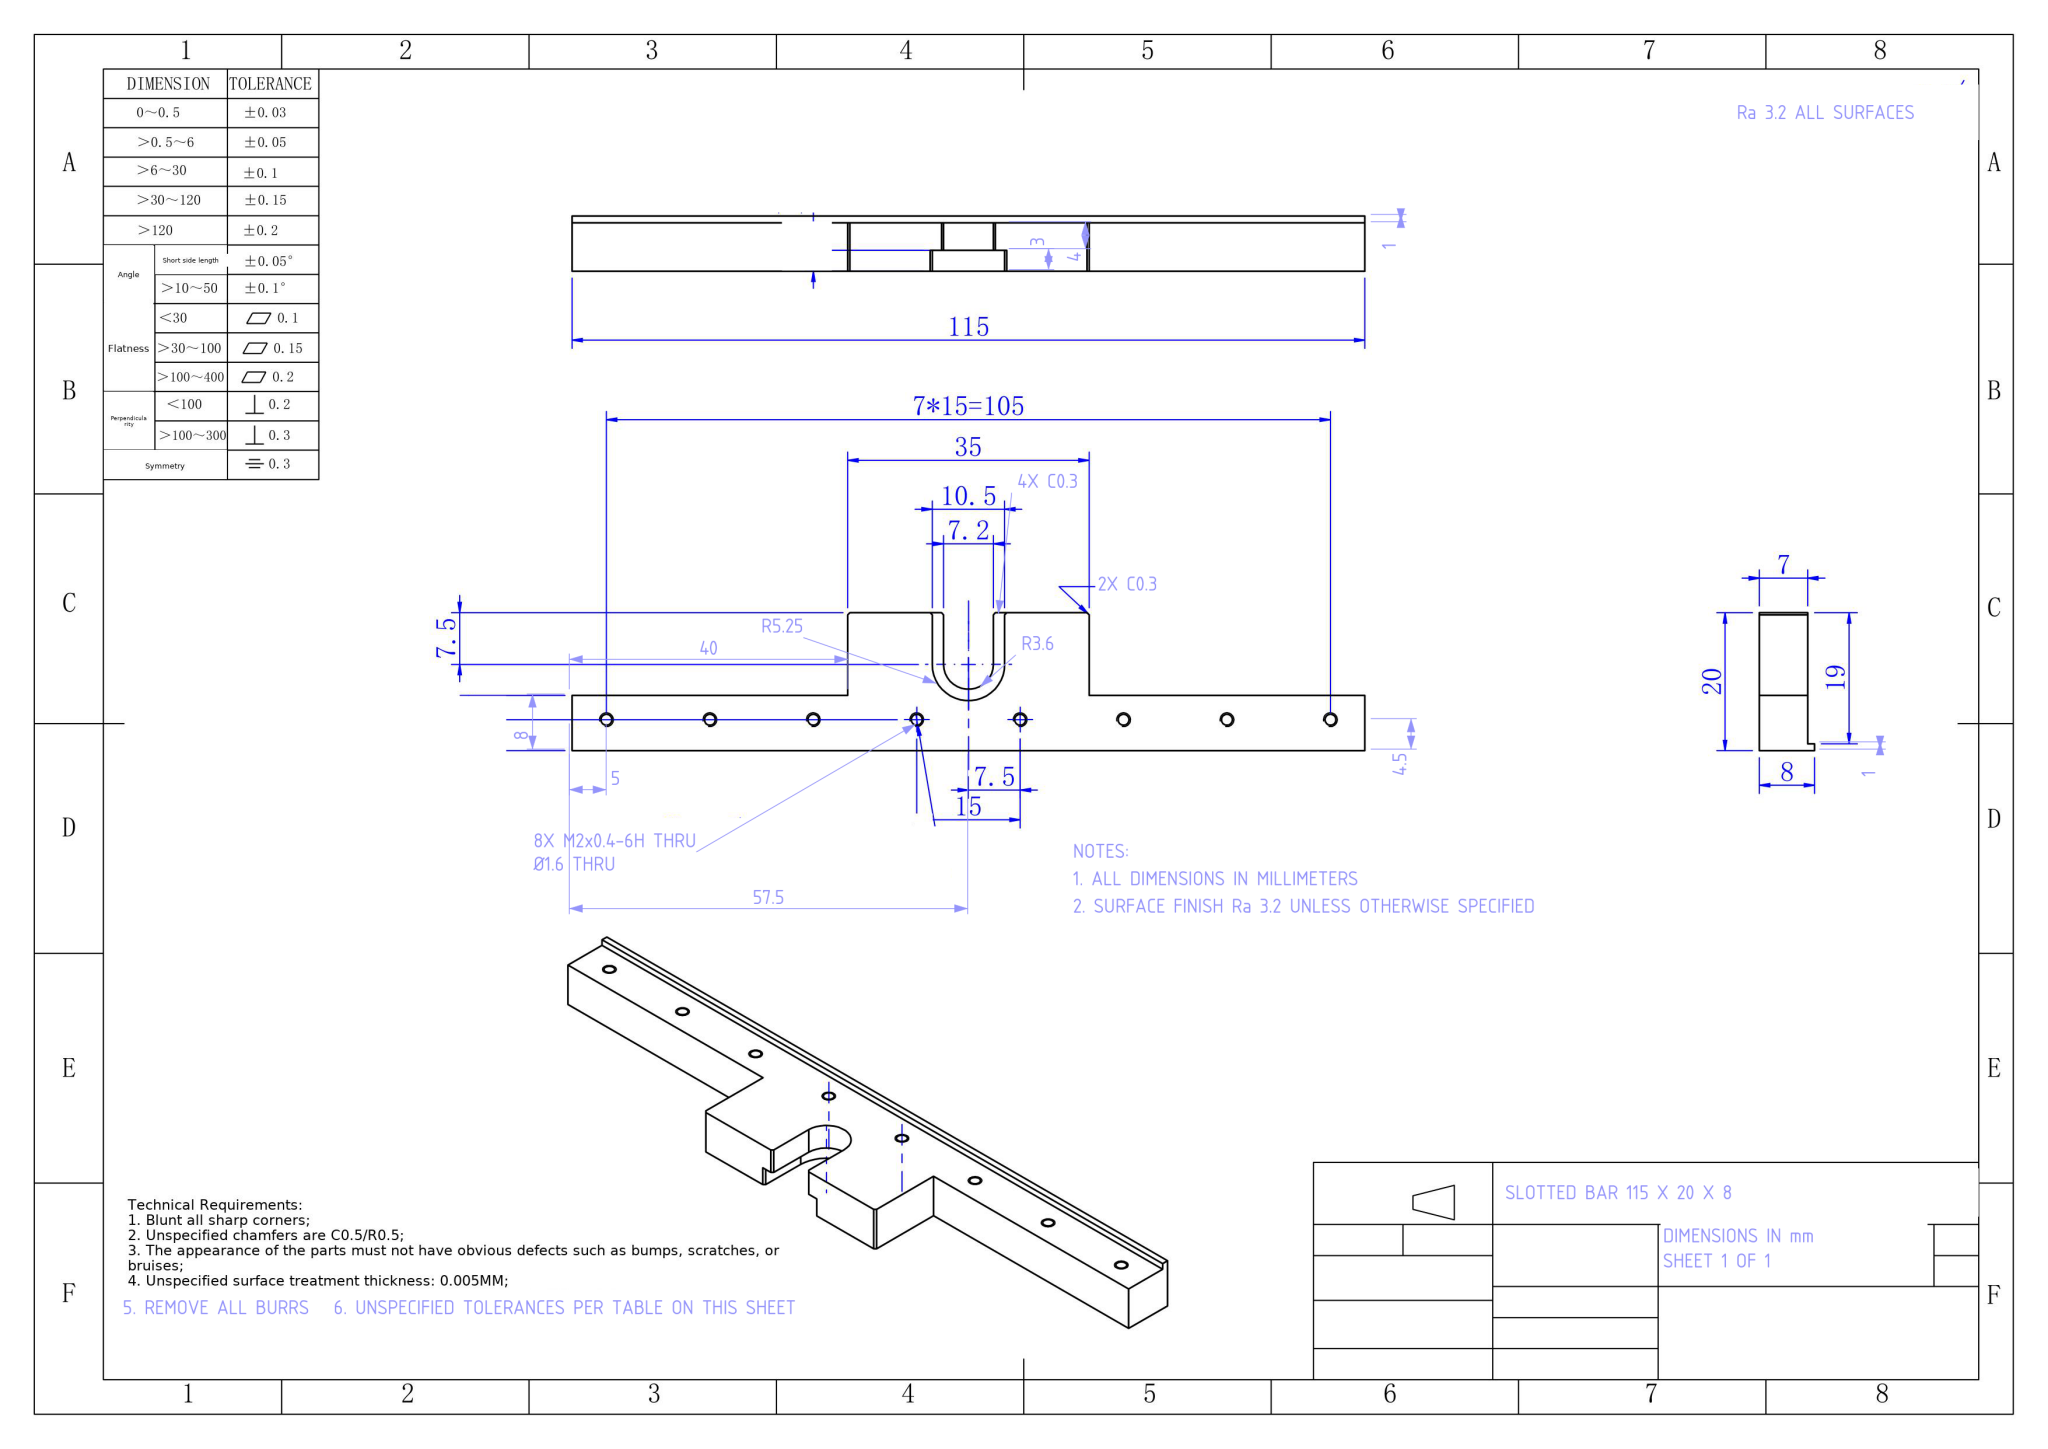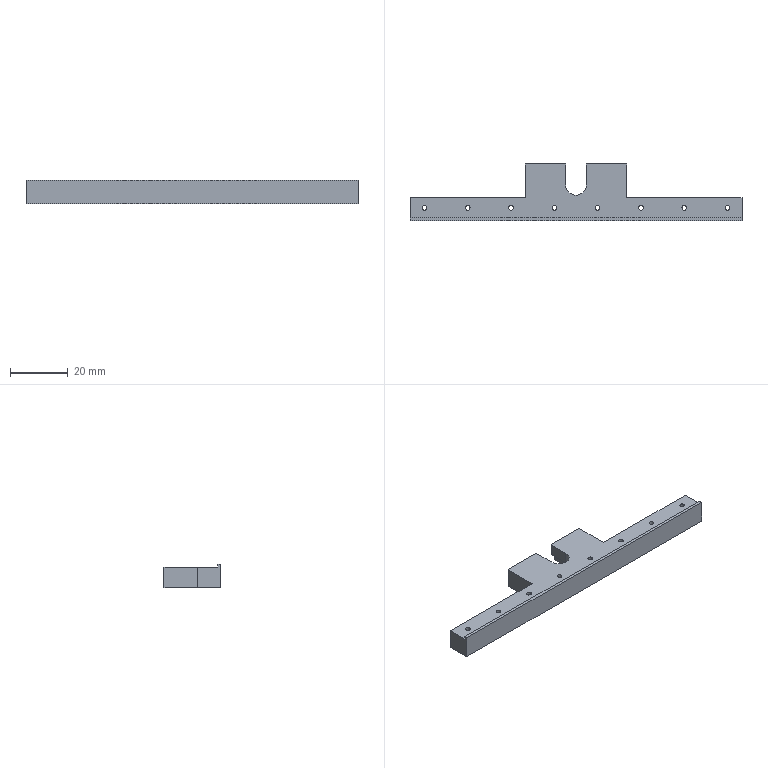Part | NX | mm | 1 solid | 42 faces | box 115 x 20 x 8 mm | volume 8718 mm3 | plane 24 | cylinder 18 | commonest cylinder face diameters 1.6 x16 7.2 x1 10.5 x1